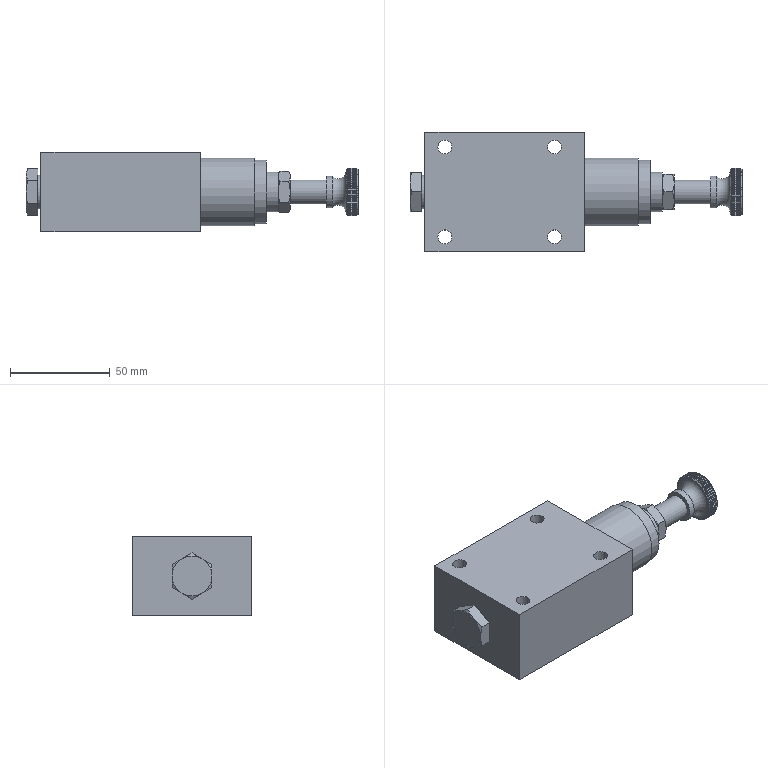Assembly | NX | mm | 11 component files | 11 solids | 506 faces | box 166.5 x 60 x 40 mm | volume 208927 mm3 | plane 249 | cone 145 | cylinder 105 | spline 5 | torus 1 | sphere 1 | commonest cylinder face diameters 24 x62 8 x4 7 x4 20 x3 12 x3 14 x3 17 x3 16 x2
Bill of materials:
unnamed part 1 | 1 |  | Hollow turned part shaped like a flanged bushing: a cylindrical hub on each side of a thin flange with a larger diameter, and a short neck with a smaller diameter between one hub and the flange. A central bore runs through the full length.
unnamed part 2 | 1 |  | Solid rectangular block. One large round bore passes through the block between the two smaller end faces. Four small round holes sit near the corners of the largest face.
GB-T6173-2000,M12x1.5 | 1 |  | Thin hexagonal prism with a centered circular through-bore, shaped like a low-profile hex nut. Both faces have conical chamfers on the hex corners, and the bore edge appears to have a small chamfer.
unnamed part 3 | 1 |  | Solid stepped cylinder: a short cylindrical head with a larger diameter joined coaxially to a longer cylindrical pin with a smaller diameter.
unnamed part 4 | 1 |  | Solid stepped shaft made of several coaxial cylindrical sections. Both ends have a smaller diameter, and a short raised collar sits near the middle.
unnamed part 5 | 1 |  | Straight solid cylindrical rod with a sphere at one end. The sphere's diameter is larger than the rod's.
unnamed part 6 | 1 |  | Stepped tubular sleeve with three outer diameters that increase along the axis. A narrow groove with a smaller diameter separates the middle and largest sections. A cylindrical bore runs through the full length.
unnamed part 7 | 1 |  | Hexagonal-head plug or bolt-like body: a hex head with chamfered corners, a short cylindrical collar under the head, and a plain cylindrical shank with a flat end.
GB806-1988,M8 | 1 |  | Knurled Nut, Collar, GB 806-1988,M8
unnamed part 8 | 1 |  | Helical coil spring with a round wire cross-section and roughly six visible coils. At least one end is closed and has a flat annular face.
unnamed part 9 | 1 |  | Flanged cylindrical pin or spacer: a long cylindrical body, a thin flange with a larger diameter, and a short cylindrical hub with a medium diameter on the other side of the flange. A small axial hole is centered on the axis.
Mates:
1. fix | valve_body 1 component
2. concentric | plug 1 edge | valve_body 1 arc
3. concentric | flow_seat 1 edge | valve_body 1 edge
4. touch align | cone_valve 1 face | flow_seat 1 face
5. touch align | spring_seat 1 face | cone_valve 1 face
6. touch align | spring_seat 1 edge | cone_valve 1 face
7. touch align | valve_stem 1 face | sleeve 1 face
8. concentric | valve_cap 1 edge | sleeve 1 edge
9. concentric | sleeve 1 edge | flow_seat 1 edge
10. concentric | valve_stem 1 edge | valve_cap 1 edge
11. touch align | cone_valve 1 face | flow_seat 1 edge
12. concentric | spring 1 edge | valve_cap 1 edge
13. concentric | GB-T6173-2000_M12x1_5 1 edge | valve_cap 1 edge
14. concentric | handle 1 edge | valve_stem 1 edge